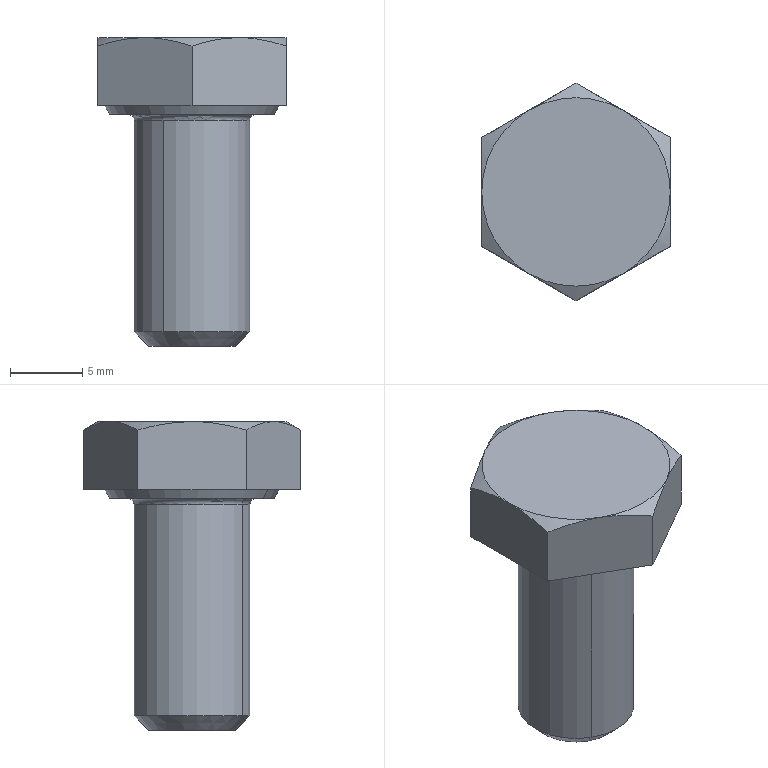Component | SolidWorks | GB_T5781-2000[HexHeadBoltFullThreadGradeCM8_16]-11 | 1 solid | 24 faces | box 13 x 15.01 x 21.3 mm | volume 1544 mm3 | cone 10 | plane 10 | cylinder 2 | torus 2 | commonest cylinder face diameters 8 x2
build123d program:
from build123d import *

# Parameters (mm, degrees)
BASE_EXTRUDE_DEPTH = 5.3
CHAMFER_2_SIZE     = 1


with BuildPart() as part:
    # Sketch1 → Base-Extrude (new body)
    with BuildSketch(Plane(origin=(0, 0, 0), x_dir=(0, 0, -1), z_dir=(1, 0, 0))):
        Polygon((6.5, 3.753), (6.5, -3.753), (0, -7.506), (-6.5, -3.753), (-6.5, 3.753), (0, 7.506), align=None)
    extrude(amount=BASE_EXTRUDE_DEPTH)

    # Sketch2 → Revolve1 (revolve)
    with BuildSketch(Plane.XY, mode=Mode.PRIVATE) as revolve1_sk:
        Polygon((0, 0), (21.3, 0), (21.3, 2.917), (21.3, 4), (5.3, 4), (0, 4), align=None)
    revolve(revolve1_sk.sketch.rotate(Axis((0, 0, 0), (-1, 0, 0)), 90), axis=Axis((0, 0, 0), (-1, 0, 0)))

    # Sketch3 → Cut-Revolve1 (revolve, cut)
    with BuildSketch(Plane.XY):
        Polygon((0, 6.5), (3.467, 12.506), (3.467, 17.506), (-10, 17.506), (-10, 6.5), align=None)
    revolve(axis=Axis((0, 0, 0), (1, 0, 0)), mode=Mode.SUBTRACT)

    # Sketch5 → Cut-Revolve2 (revolve, cut)
    with BuildSketch(Plane.XY):
        Polygon((5.3, 6.5), (1.833, 12.506), (1.833, 17.506), (11.833, 17.506), (11.833, 6.5), align=None)
    revolve(axis=Axis((0, 0, 0), (1, 0, 0)), mode=Mode.SUBTRACT)

    # Sketch4 → Cut-Revolve3 (revolve, cut)
    with BuildSketch(Plane.XY, mode=Mode.PRIVATE) as cut_revolve3_sk:
        Polygon((5.3, 5.677), (4.7, 6.024), (4.7, 17.506), (5.3, 17.506), align=None)
    revolve(cut_revolve3_sk.sketch.rotate(Axis((0, 0, 0), (1, 0, 0)), 90), axis=Axis((0, 0, 0), (1, 0, 0)), mode=Mode.SUBTRACT)

    # Chamfer 2
    chamfer_2_edges = [part.edges().sort_by_distance(p)[0] for p in [
        (21.3, 0, 4),
    ]]
    chamfer(chamfer_2_edges, length=CHAMFER_2_SIZE)

    # Sketch9 → Revolve1_2 (revolve)
    with BuildSketch(Plane.XY, mode=Mode.PRIVATE) as revolve1_2_sk:
        with BuildLine():
            Line((5.3, 4.4), (5.3, 4))
            Line((5.3, 4), (5.7, 4))
            ThreePointArc((5.7, 4), (5.417, 4.117), (5.3, 4.4))
        make_face()
    revolve(revolve1_2_sk.sketch.rotate(Axis((0, 0, 0), (1, 0, 0)), 90), axis=Axis((0, 0, 0), (1, 0, 0)))


solid = part.part

# Placed as in the assembly
solid = solid.moved(Location((24.99, 1.047, 168.3), (0, 90, 0)))
STEP:
#1=CARTESIAN_POINT('',(0.9051,-0.09515,6.402));
#2=VERTEX_POINT('',#1);
#3=CARTESIAN_POINT('',(1.063,0.1776,6.402));
#4=VERTEX_POINT('',#3);
#5=CARTESIAN_POINT('',(0.9839,0.04123,6.402));
#6=DIRECTION('',(-0.,-0.,1.));
#7=DIRECTION('',(-0.5,-0.866,-0.));
#8=AXIS2_PLACEMENT_3D('',#5,#6,#7);
#9=CIRCLE('',#8,0.1575);
#10=EDGE_CURVE('',#2,#4,#9,.T.);
#11=ORIENTED_EDGE('',*,*,#10,.F.);
#12=CARTESIAN_POINT('',(0.9051,-0.09515,5.827));
#13=VERTEX_POINT('',#12);
#14=CARTESIAN_POINT('',(0.9051,-0.09515,6.626));
#15=DIRECTION('',(0.,0.,-1.));
#16=VECTOR('',#15,39.37);
#17=LINE('',#14,#16);
#18=EDGE_CURVE('',#2,#13,#17,.T.);
#19=ORIENTED_EDGE('',*,*,#18,.T.);
#20=CARTESIAN_POINT('',(1.063,0.1776,5.827));
#21=VERTEX_POINT('',#20);
#22=CARTESIAN_POINT('',(0.9839,0.04123,5.827));
#23=DIRECTION('',(-0.,-0.,1.));
#24=DIRECTION('',(0.5,0.866,0.));
#25=AXIS2_PLACEMENT_3D('',#22,#23,#24);
#26=CIRCLE('',#25,0.1575);
#27=EDGE_CURVE('',#13,#21,#26,.T.);
#28=ORIENTED_EDGE('',*,*,#27,.T.);
#29=CARTESIAN_POINT('',(1.063,0.1776,6.626));
#30=DIRECTION('',(0.,0.,-1.));
#31=VECTOR('',#30,39.37);
#32=LINE('',#29,#31);
#33=EDGE_CURVE('',#4,#21,#32,.T.);
#34=ORIENTED_EDGE('',*,*,#33,.F.);
#35=EDGE_LOOP('',(#11,#19,#28,#34));
#36=FACE_OUTER_BOUND('',#35,.T.);
#37=CARTESIAN_POINT('',(0.9839,0.04123,6.626));
#38=DIRECTION('',(0.,0.,-1.));
#39=DIRECTION('',(0.5,0.866,0.));
#40=AXIS2_PLACEMENT_3D('',#37,#38,#39);
#41=CYLINDRICAL_SURFACE('',#40,0.1575);
#42=ADVANCED_FACE('',(#36),#41,.T.);
#43=CARTESIAN_POINT('',(1.043,0.1435,5.787));
#44=VERTEX_POINT('',#43);
#45=CARTESIAN_POINT('',(0.9248,-0.06106,5.787));
#46=VERTEX_POINT('',#45);
#47=CARTESIAN_POINT('',(0.9839,0.04123,5.787));
#48=DIRECTION('',(0.,0.,-1.));
#49=DIRECTION('',(0.5,0.866,0.));
#50=AXIS2_PLACEMENT_3D('',#47,#48,#49);
#51=CIRCLE('',#50,0.1181);
#52=EDGE_CURVE('',#44,#46,#51,.T.);
#53=ORIENTED_EDGE('',*,*,#52,.F.);
#54=CARTESIAN_POINT('',(1.043,0.1435,5.787));
#55=DIRECTION('',(0.3536,0.6124,0.7071));
#56=VECTOR('',#55,39.37);
#57=LINE('',#54,#56);
#58=EDGE_CURVE('',#44,#21,#57,.T.);
#59=ORIENTED_EDGE('',*,*,#58,.T.);
#60=ORIENTED_EDGE('',*,*,#27,.F.);
#61=CARTESIAN_POINT('',(0.9248,-0.06106,5.787));
#62=DIRECTION('',(-0.3536,-0.6124,0.7071));
#63=VECTOR('',#62,39.37);
#64=LINE('',#61,#63);
#65=EDGE_CURVE('',#46,#13,#64,.T.);
#66=ORIENTED_EDGE('',*,*,#65,.F.);
#67=EDGE_LOOP('',(#53,#59,#60,#66));
#68=FACE_OUTER_BOUND('',#67,.T.);
#69=CARTESIAN_POINT('',(0.9839,0.04123,5.787));
#70=DIRECTION('',(-0.,-0.,1.));
#71=DIRECTION('',(-0.5,-0.866,0.));
#72=AXIS2_PLACEMENT_3D('',#69,#70,#71);
#73=CONICAL_SURFACE('',#72,0.1181,0.7854);
#74=ADVANCED_FACE('',(#68),#73,.T.);
#75=CARTESIAN_POINT('',(1.07,0.1913,6.417));
#76=VERTEX_POINT('',#75);
#77=CARTESIAN_POINT('',(0.8972,-0.1088,6.417));
#78=VERTEX_POINT('',#77);
#79=CARTESIAN_POINT('',(0.9839,0.04123,6.417));
#80=DIRECTION('',(-0.,-0.,1.));
#81=DIRECTION('',(-0.5,-0.866,-0.));
#82=AXIS2_PLACEMENT_3D('',#79,#80,#81);
#83=CIRCLE('',#82,0.1732);
#84=EDGE_CURVE('',#76,#78,#83,.T.);
#85=ORIENTED_EDGE('',*,*,#84,.F.);
#86=CARTESIAN_POINT('',(1.07,0.1913,6.402));
#87=DIRECTION('',(0.866,-0.5,-0.));
#88=DIRECTION('',(0.5,0.866,0.));
#89=AXIS2_PLACEMENT_3D('',#86,#87,#88);
#90=CIRCLE('',#89,0.01575);
#91=EDGE_CURVE('',#76,#4,#90,.T.);
#92=ORIENTED_EDGE('',*,*,#91,.T.);
#93=CARTESIAN_POINT('',(0.9839,0.04123,6.402));
#94=DIRECTION('',(-0.,-0.,1.));
#95=DIRECTION('',(-0.5,-0.866,-0.));
#96=AXIS2_PLACEMENT_3D('',#93,#94,#95);
#97=CIRCLE('',#96,0.1575);
#98=EDGE_CURVE('',#4,#2,#97,.T.);
#99=ORIENTED_EDGE('',*,*,#98,.T.);
#100=CARTESIAN_POINT('',(0.8972,-0.1088,6.402));
#101=DIRECTION('',(-0.866,0.5,0.));
#102=DIRECTION('',(-0.5,-0.866,0.));
#103=AXIS2_PLACEMENT_3D('',#100,#101,#102);
#104=CIRCLE('',#103,0.01575);
#105=EDGE_CURVE('',#78,#2,#104,.T.);
#106=ORIENTED_EDGE('',*,*,#105,.F.);
#107=EDGE_LOOP('',(#85,#92,#99,#106));
#108=FACE_OUTER_BOUND('',#107,.T.);
#109=CARTESIAN_POINT('',(0.9839,0.04123,6.402));
#110=DIRECTION('',(-0.,-0.,1.));
#111=DIRECTION('',(-0.5,-0.866,-0.));
#112=AXIS2_PLACEMENT_3D('',#109,#110,#111);
#113=TOROIDAL_SURFACE('',#112,0.1732,0.01575);
#114=ADVANCED_FACE('',(#108),#113,.F.);
#115=CARTESIAN_POINT('',(0.8721,-0.1523,6.417));
#116=VERTEX_POINT('',#115);
#117=CARTESIAN_POINT('',(1.096,0.2348,6.417));
#118=VERTEX_POINT('',#117);
#119=CARTESIAN_POINT('',(0.9839,0.04123,6.417));
#120=DIRECTION('',(-0.,-0.,1.));
#121=DIRECTION('',(-0.5,-0.866,-0.));
#122=AXIS2_PLACEMENT_3D('',#119,#120,#121);
#123=CIRCLE('',#122,0.2235);
#124=EDGE_CURVE('',#116,#118,#123,.T.);
#125=ORIENTED_EDGE('',*,*,#124,.T.);
#126=CARTESIAN_POINT('',(1.102,0.2466,6.441));
#127=VERTEX_POINT('',#126);
#128=CARTESIAN_POINT('',(1.102,0.2466,6.441));
#129=DIRECTION('',(0.25,0.433,0.866));
#130=VECTOR('',#129,39.37);
#131=LINE('',#128,#130);
#132=EDGE_CURVE('',#118,#127,#131,.T.);
#133=ORIENTED_EDGE('',*,*,#132,.T.);
#134=CARTESIAN_POINT('',(0.8653,-0.1641,6.441));
#135=VERTEX_POINT('',#134);
#136=CARTESIAN_POINT('',(0.9839,0.04123,6.441));
#137=DIRECTION('',(-0.,-0.,1.));
#138=DIRECTION('',(-0.5,-0.866,-0.));
#139=AXIS2_PLACEMENT_3D('',#136,#137,#138);
#140=CIRCLE('',#139,0.2372);
#141=EDGE_CURVE('',#135,#127,#140,.T.);
#142=ORIENTED_EDGE('',*,*,#141,.F.);
#143=CARTESIAN_POINT('',(0.8653,-0.1641,6.441));
#144=DIRECTION('',(-0.25,-0.433,0.866));
#145=VECTOR('',#144,39.37);
#146=LINE('',#143,#145);
#147=EDGE_CURVE('',#116,#135,#146,.T.);
#148=ORIENTED_EDGE('',*,*,#147,.F.);
#149=EDGE_LOOP('',(#125,#133,#142,#148));
#150=FACE_OUTER_BOUND('',#149,.T.);
#151=CARTESIAN_POINT('',(0.9839,0.04123,6.441));
#152=DIRECTION('',(-0.,-0.,1.));
#153=DIRECTION('',(-0.5,-0.866,-0.));
#154=AXIS2_PLACEMENT_3D('',#151,#152,#153);
#155=CONICAL_SURFACE('',#154,0.2372,0.5236);
#156=ADVANCED_FACE('',(#150),#155,.T.);
#157=ORIENTED_EDGE('',*,*,#124,.F.);
#158=CARTESIAN_POINT('',(0.9839,0.04123,6.417));
#159=DIRECTION('',(-0.,-0.,1.));
#160=DIRECTION('',(-0.5,-0.866,-0.));
#161=AXIS2_PLACEMENT_3D('',#158,#159,#160);
#162=CIRCLE('',#161,0.2235);
#163=EDGE_CURVE('',#118,#116,#162,.T.);
#164=ORIENTED_EDGE('',*,*,#163,.F.);
#165=EDGE_LOOP('',(#157,#164));
#166=FACE_OUTER_BOUND('',#165,.T.);
#167=CARTESIAN_POINT('',(0.9839,0.04123,6.417));
#168=DIRECTION('',(-0.,-0.,1.));
#169=DIRECTION('',(-0.5,-0.866,-0.));
#170=AXIS2_PLACEMENT_3D('',#167,#168,#169);
#171=CIRCLE('',#170,0.1732);
#172=EDGE_CURVE('',#78,#76,#171,.T.);
#173=ORIENTED_EDGE('',*,*,#172,.T.);
#174=ORIENTED_EDGE('',*,*,#84,.T.);
#175=EDGE_LOOP('',(#173,#174));
#176=FACE_BOUND('',#175,.T.);
#177=CARTESIAN_POINT('',(1.24,-0.1065,6.417));
#178=DIRECTION('',(0.,0.,-1.));
#179=DIRECTION('',(0.5,0.866,0.));
#180=AXIS2_PLACEMENT_3D('',#177,#178,#179);
#181=PLANE('',#180);
#182=ADVANCED_FACE('',(#166,#176),#181,.T.);
#183=CARTESIAN_POINT('',(1.24,0.189,6.441));
#184=VERTEX_POINT('',#183);
#185=CARTESIAN_POINT('',(1.24,-0.1065,6.441));
#186=VERTEX_POINT('',#185);
#187=CARTESIAN_POINT('',(1.24,0.189,6.441));
#188=DIRECTION('',(0.,-1.,-0.));
#189=VECTOR('',#188,39.37);
#190=LINE('',#187,#189);
#191=EDGE_CURVE('',#184,#186,#190,.T.);
#192=ORIENTED_EDGE('',*,*,#191,.F.);
#193=CARTESIAN_POINT('',(1.24,0.189,6.603));
#194=VERTEX_POINT('',#193);
#195=CARTESIAN_POINT('',(1.24,0.189,6.417));
#196=DIRECTION('',(-0.,-0.,1.));
#197=VECTOR('',#196,39.37);
#198=LINE('',#195,#197);
#199=EDGE_CURVE('',#184,#194,#198,.T.);
#200=ORIENTED_EDGE('',*,*,#199,.T.);
#201=CARTESIAN_POINT('',(1.24,0.04123,6.626));
#202=VERTEX_POINT('',#201);
#203=CARTESIAN_POINT('',(1.24,0.04123,6.626));
#204=CARTESIAN_POINT('',(1.24,0.05377,6.626));
#205=CARTESIAN_POINT('',(1.24,0.06637,6.625));
#206=CARTESIAN_POINT('',(1.24,0.09128,6.623));
#207=CARTESIAN_POINT('',(1.24,0.1037,6.622));
#208=CARTESIAN_POINT('',(1.24,0.1406,6.616));
#209=CARTESIAN_POINT('',(1.24,0.1649,6.61));
#210=CARTESIAN_POINT('',(1.24,0.189,6.603));
#211=B_SPLINE_CURVE_WITH_KNOTS('',3,(#203,#204,#205,#206,#207,#208,#209,#210),.UNSPECIFIED.,.F.,.F.,(4,2,2,4),(0.003797,0.004743,0.005689,0.00758),.UNSPECIFIED.);
#212=EDGE_CURVE('',#202,#194,#211,.T.);
#213=ORIENTED_EDGE('',*,*,#212,.F.);
#214=CARTESIAN_POINT('',(1.24,-0.1065,6.603));
#215=VERTEX_POINT('',#214);
#216=CARTESIAN_POINT('',(1.24,-0.1065,6.603));
#217=CARTESIAN_POINT('',(1.24,-0.08235,6.61));
#218=CARTESIAN_POINT('',(1.24,-0.058,6.616));
#219=CARTESIAN_POINT('',(1.24,-0.008799,6.624));
#220=CARTESIAN_POINT('',(1.24,0.01606,6.626));
#221=CARTESIAN_POINT('',(1.24,0.04123,6.626));
#222=B_SPLINE_CURVE_WITH_KNOTS('',3,(#216,#217,#218,#219,#220,#221),.UNSPECIFIED.,.F.,.F.,(4,2,4),(0.00000024,0.001899,0.003797),.UNSPECIFIED.);
#223=EDGE_CURVE('',#215,#202,#222,.T.);
#224=ORIENTED_EDGE('',*,*,#223,.F.);
#225=CARTESIAN_POINT('',(1.24,-0.1065,6.417));
#226=DIRECTION('',(-0.,-0.,1.));
#227=VECTOR('',#226,39.37);
#228=LINE('',#225,#227);
#229=EDGE_CURVE('',#186,#215,#228,.T.);
#230=ORIENTED_EDGE('',*,*,#229,.F.);
#231=EDGE_LOOP('',(#192,#200,#213,#224,#230));
#232=FACE_OUTER_BOUND('',#231,.T.);
#233=CARTESIAN_POINT('',(1.24,0.189,6.417));
#234=DIRECTION('',(-1.,-0.,-0.));
#235=DIRECTION('',(-0.,1.,0.));
#236=AXIS2_PLACEMENT_3D('',#233,#234,#235);
#237=PLANE('',#236);
#238=ADVANCED_FACE('',(#232),#237,.F.);
#239=CARTESIAN_POINT('',(0.9839,-0.2543,6.441));
#240=VERTEX_POINT('',#239);
#241=CARTESIAN_POINT('',(1.24,-0.1065,6.441));
#242=DIRECTION('',(-0.866,-0.5,-0.));
#243=VECTOR('',#242,39.37);
#244=LINE('',#241,#243);
#245=EDGE_CURVE('',#186,#240,#244,.T.);
#246=ORIENTED_EDGE('',*,*,#245,.F.);
#247=ORIENTED_EDGE('',*,*,#229,.T.);
#248=CARTESIAN_POINT('',(1.112,-0.1804,6.626));
#249=VERTEX_POINT('',#248);
#250=CARTESIAN_POINT('',(1.112,-0.1804,6.626));
#251=CARTESIAN_POINT('',(1.123,-0.1741,6.626));
#252=CARTESIAN_POINT('',(1.134,-0.1678,6.625));
#253=CARTESIAN_POINT('',(1.155,-0.1554,6.623));
#254=CARTESIAN_POINT('',(1.166,-0.1492,6.622));
#255=CARTESIAN_POINT('',(1.198,-0.1307,6.616));
#256=CARTESIAN_POINT('',(1.219,-0.1186,6.61));
#257=CARTESIAN_POINT('',(1.24,-0.1065,6.603));
#258=B_SPLINE_CURVE_WITH_KNOTS('',3,(#250,#251,#252,#253,#254,#255,#256,#257),.UNSPECIFIED.,.F.,.F.,(4,2,2,4),(0.003797,0.004743,0.005689,0.00758),.UNSPECIFIED.);
#259=EDGE_CURVE('',#249,#215,#258,.T.);
#260=ORIENTED_EDGE('',*,*,#259,.F.);
#261=CARTESIAN_POINT('',(0.9839,-0.2543,6.603));
#262=VERTEX_POINT('',#261);
#263=CARTESIAN_POINT('',(0.9839,-0.2543,6.603));
#264=CARTESIAN_POINT('',(1.005,-0.2422,6.61));
#265=CARTESIAN_POINT('',(1.026,-0.23,6.616));
#266=CARTESIAN_POINT('',(1.068,-0.2054,6.624));
#267=CARTESIAN_POINT('',(1.09,-0.193,6.626));
#268=CARTESIAN_POINT('',(1.112,-0.1804,6.626));
#269=B_SPLINE_CURVE_WITH_KNOTS('',3,(#263,#264,#265,#266,#267,#268),.UNSPECIFIED.,.F.,.F.,(4,2,4),(0.00000024,0.001899,0.003797),.UNSPECIFIED.);
#270=EDGE_CURVE('',#262,#249,#269,.T.);
#271=ORIENTED_EDGE('',*,*,#270,.F.);
#272=CARTESIAN_POINT('',(0.9839,-0.2543,6.417));
#273=DIRECTION('',(-0.,-0.,1.));
#274=VECTOR('',#273,39.37);
#275=LINE('',#272,#274);
#276=EDGE_CURVE('',#240,#262,#275,.T.);
#277=ORIENTED_EDGE('',*,*,#276,.F.);
#278=EDGE_LOOP('',(#246,#247,#260,#271,#277));
#279=FACE_OUTER_BOUND('',#278,.T.);
#280=CARTESIAN_POINT('',(1.24,-0.1065,6.417));
#281=DIRECTION('',(-0.5,0.866,0.));
#282=DIRECTION('',(0.866,0.5,0.));
#283=AXIS2_PLACEMENT_3D('',#280,#281,#282);
#284=PLANE('',#283);
#285=ADVANCED_FACE('',(#279),#284,.F.);
#286=CARTESIAN_POINT('',(0.728,-0.1065,6.441));
#287=VERTEX_POINT('',#286);
#288=CARTESIAN_POINT('',(0.9839,-0.2543,6.441));
#289=DIRECTION('',(-0.866,0.5,0.));
#290=VECTOR('',#289,39.37);
#291=LINE('',#288,#290);
#292=EDGE_CURVE('',#240,#287,#291,.T.);
#293=ORIENTED_EDGE('',*,*,#292,.F.);
#294=ORIENTED_EDGE('',*,*,#276,.T.);
#295=CARTESIAN_POINT('',(0.8559,-0.1804,6.626));
#296=VERTEX_POINT('',#295);
#297=CARTESIAN_POINT('',(0.8559,-0.1804,6.626));
#298=CARTESIAN_POINT('',(0.8776,-0.1929,6.626));
#299=CARTESIAN_POINT('',(0.8995,-0.2056,6.624));
#300=CARTESIAN_POINT('',(0.9422,-0.2302,6.616));
#301=CARTESIAN_POINT('',(0.9632,-0.2423,6.61));
#302=CARTESIAN_POINT('',(0.9839,-0.2543,6.603));
#303=B_SPLINE_CURVE_WITH_KNOTS('',3,(#297,#298,#299,#300,#301,#302),.UNSPECIFIED.,.F.,.F.,(4,2,4),(0.01067,0.01257,0.01447),.UNSPECIFIED.);
#304=EDGE_CURVE('',#296,#262,#303,.T.);
#305=ORIENTED_EDGE('',*,*,#304,.F.);
#306=CARTESIAN_POINT('',(0.728,-0.1065,6.603));
#307=VERTEX_POINT('',#306);
#308=CARTESIAN_POINT('',(0.728,-0.1065,6.603));
#309=CARTESIAN_POINT('',(0.7488,-0.1185,6.61));
#310=CARTESIAN_POINT('',(0.7701,-0.1308,6.616));
#311=CARTESIAN_POINT('',(0.8128,-0.1555,6.624));
#312=CARTESIAN_POINT('',(0.8343,-0.1679,6.626));
#313=CARTESIAN_POINT('',(0.8559,-0.1804,6.626));
#314=B_SPLINE_CURVE_WITH_KNOTS('',3,(#308,#309,#310,#311,#312,#313),.UNSPECIFIED.,.F.,.F.,(4,2,4),(0.006874,0.008773,0.01067),.UNSPECIFIED.);
#315=EDGE_CURVE('',#307,#296,#314,.T.);
#316=ORIENTED_EDGE('',*,*,#315,.F.);
#317=CARTESIAN_POINT('',(0.728,-0.1065,6.417));
#318=DIRECTION('',(-0.,-0.,1.));
#319=VECTOR('',#318,39.37);
#320=LINE('',#317,#319);
#321=EDGE_CURVE('',#287,#307,#320,.T.);
#322=ORIENTED_EDGE('',*,*,#321,.F.);
#323=EDGE_LOOP('',(#293,#294,#305,#316,#322));
#324=FACE_OUTER_BOUND('',#323,.T.);
#325=CARTESIAN_POINT('',(0.9839,-0.2543,6.417));
#326=DIRECTION('',(0.5,0.866,0.));
#327=DIRECTION('',(0.866,-0.5,-0.));
#328=AXIS2_PLACEMENT_3D('',#325,#326,#327);
#329=PLANE('',#328);
#330=ADVANCED_FACE('',(#324),#329,.F.);
#331=CARTESIAN_POINT('',(0.728,0.189,6.441));
#332=VERTEX_POINT('',#331);
#333=CARTESIAN_POINT('',(0.728,0.189,6.441));
#334=DIRECTION('',(-0.,1.,0.));
#335=VECTOR('',#334,39.37);
#336=LINE('',#333,#335);
#337=EDGE_CURVE('',#287,#332,#336,.T.);
#338=ORIENTED_EDGE('',*,*,#337,.F.);
#339=ORIENTED_EDGE('',*,*,#321,.T.);
#340=CARTESIAN_POINT('',(0.728,0.04123,6.626));
#341=VERTEX_POINT('',#340);
#342=CARTESIAN_POINT('',(0.728,0.04123,6.626));
#343=CARTESIAN_POINT('',(0.728,0.02869,6.626));
#344=CARTESIAN_POINT('',(0.728,0.0161,6.625));
#345=CARTESIAN_POINT('',(0.728,-0.008818,6.623));
#346=CARTESIAN_POINT('',(0.728,-0.02119,6.622));
#347=CARTESIAN_POINT('',(0.728,-0.0581,6.616));
#348=CARTESIAN_POINT('',(0.728,-0.08241,6.61));
#349=CARTESIAN_POINT('',(0.728,-0.1065,6.603));
#350=B_SPLINE_CURVE_WITH_KNOTS('',3,(#342,#343,#344,#345,#346,#347,#348,#349),.UNSPECIFIED.,.F.,.F.,(4,2,2,4),(0.003797,0.004743,0.005689,0.00758),.UNSPECIFIED.);
#351=EDGE_CURVE('',#341,#307,#350,.T.);
#352=ORIENTED_EDGE('',*,*,#351,.F.);
#353=CARTESIAN_POINT('',(0.728,0.189,6.603));
#354=VERTEX_POINT('',#353);
#355=CARTESIAN_POINT('',(0.728,0.189,6.603));
#356=CARTESIAN_POINT('',(0.728,0.1648,6.61));
#357=CARTESIAN_POINT('',(0.728,0.1405,6.616));
#358=CARTESIAN_POINT('',(0.728,0.09126,6.624));
#359=CARTESIAN_POINT('',(0.728,0.0664,6.626));
#360=CARTESIAN_POINT('',(0.728,0.04123,6.626));
#361=B_SPLINE_CURVE_WITH_KNOTS('',3,(#355,#356,#357,#358,#359,#360),.UNSPECIFIED.,.F.,.F.,(4,2,4),(0.00000024,0.001899,0.003797),.UNSPECIFIED.);
#362=EDGE_CURVE('',#354,#341,#361,.T.);
#363=ORIENTED_EDGE('',*,*,#362,.F.);
#364=CARTESIAN_POINT('',(0.728,0.189,6.417));
#365=DIRECTION('',(-0.,-0.,1.));
#366=VECTOR('',#365,39.37);
#367=LINE('',#364,#366);
#368=EDGE_CURVE('',#332,#354,#367,.T.);
#369=ORIENTED_EDGE('',*,*,#368,.F.);
#370=EDGE_LOOP('',(#338,#339,#352,#363,#369));
#371=FACE_OUTER_BOUND('',#370,.T.);
#372=CARTESIAN_POINT('',(0.728,0.189,6.417));
#373=DIRECTION('',(1.,0.,0.));
#374=DIRECTION('',(0.,-1.,-0.));
#375=AXIS2_PLACEMENT_3D('',#372,#373,#374);
#376=PLANE('',#375);
#377=ADVANCED_FACE('',(#371),#376,.F.);
#378=CARTESIAN_POINT('',(0.9839,0.3367,6.441));
#379=VERTEX_POINT('',#378);
#380=CARTESIAN_POINT('',(0.9839,0.3367,6.441));
#381=DIRECTION('',(0.866,0.5,0.));
#382=VECTOR('',#381,39.37);
#383=LINE('',#380,#382);
#384=EDGE_CURVE('',#332,#379,#383,.T.);
#385=ORIENTED_EDGE('',*,*,#384,.F.);
#386=ORIENTED_EDGE('',*,*,#368,.T.);
#387=CARTESIAN_POINT('',(0.8559,0.2629,6.626));
#388=VERTEX_POINT('',#387);
#389=CARTESIAN_POINT('',(0.8559,0.2629,6.626));
#390=CARTESIAN_POINT('',(0.845,0.2566,6.626));
#391=CARTESIAN_POINT('',(0.8341,0.2503,6.625));
#392=CARTESIAN_POINT('',(0.8126,0.2378,6.623));
#393=CARTESIAN_POINT('',(0.8018,0.2316,6.622));
#394=CARTESIAN_POINT('',(0.7699,0.2132,6.616));
#395=CARTESIAN_POINT('',(0.7488,0.201,6.61));
#396=CARTESIAN_POINT('',(0.728,0.189,6.603));
#397=B_SPLINE_CURVE_WITH_KNOTS('',3,(#389,#390,#391,#392,#393,#394,#395,#396),.UNSPECIFIED.,.F.,.F.,(4,2,2,4),(0.003797,0.004743,0.005689,0.00758),.UNSPECIFIED.);
#398=EDGE_CURVE('',#388,#354,#397,.T.);
#399=ORIENTED_EDGE('',*,*,#398,.F.);
#400=CARTESIAN_POINT('',(0.9839,0.3367,6.603));
#401=VERTEX_POINT('',#400);
#402=CARTESIAN_POINT('',(0.9839,0.3367,6.603));
#403=CARTESIAN_POINT('',(0.9629,0.3246,6.61));
#404=CARTESIAN_POINT('',(0.9418,0.3125,6.616));
#405=CARTESIAN_POINT('',(0.8992,0.2879,6.624));
#406=CARTESIAN_POINT('',(0.8777,0.2754,6.626));
#407=CARTESIAN_POINT('',(0.8559,0.2629,6.626));
#408=B_SPLINE_CURVE_WITH_KNOTS('',3,(#402,#403,#404,#405,#406,#407),.UNSPECIFIED.,.F.,.F.,(4,2,4),(0.00000024,0.001899,0.003797),.UNSPECIFIED.);
#409=EDGE_CURVE('',#401,#388,#408,.T.);
#410=ORIENTED_EDGE('',*,*,#409,.F.);
#411=CARTESIAN_POINT('',(0.9839,0.3367,6.417));
#412=DIRECTION('',(-0.,-0.,1.));
#413=VECTOR('',#412,39.37);
#414=LINE('',#411,#413);
#415=EDGE_CURVE('',#379,#401,#414,.T.);
#416=ORIENTED_EDGE('',*,*,#415,.F.);
#417=EDGE_LOOP('',(#385,#386,#399,#410,#416));
#418=FACE_OUTER_BOUND('',#417,.T.);
#419=CARTESIAN_POINT('',(0.9839,0.3367,6.417));
#420=DIRECTION('',(0.5,-0.866,-0.));
#421=DIRECTION('',(-0.866,-0.5,-0.));
#422=AXIS2_PLACEMENT_3D('',#419,#420,#421);
#423=PLANE('',#422);
#424=ADVANCED_FACE('',(#418),#423,.F.);
#425=CARTESIAN_POINT('',(1.24,0.189,6.441));
#426=DIRECTION('',(0.866,-0.5,-0.));
#427=VECTOR('',#426,39.37);
#428=LINE('',#425,#427);
#429=EDGE_CURVE('',#379,#184,#428,.T.);
#430=ORIENTED_EDGE('',*,*,#429,.F.);
#431=ORIENTED_EDGE('',*,*,#415,.T.);
#432=CARTESIAN_POINT('',(1.112,0.2629,6.626));
#433=VERTEX_POINT('',#432);
#434=CARTESIAN_POINT('',(1.112,0.2629,6.626));
#435=CARTESIAN_POINT('',(1.09,0.2753,6.626));
#436=CARTESIAN_POINT('',(1.069,0.2877,6.624));
#437=CARTESIAN_POINT('',(1.026,0.3124,6.616));
#438=CARTESIAN_POINT('',(1.005,0.3247,6.61));
#439=CARTESIAN_POINT('',(0.9839,0.3367,6.603));
#440=B_SPLINE_CURVE_WITH_KNOTS('',3,(#434,#435,#436,#437,#438,#439),.UNSPECIFIED.,.F.,.F.,(4,2,4),(0.02294,0.02484,0.02674),.UNSPECIFIED.);
#441=EDGE_CURVE('',#433,#401,#440,.T.);
#442=ORIENTED_EDGE('',*,*,#441,.F.);
#443=CARTESIAN_POINT('',(1.24,0.189,6.603));
#444=CARTESIAN_POINT('',(1.219,0.2009,6.61));
#445=CARTESIAN_POINT('',(1.198,0.213,6.616));
#446=CARTESIAN_POINT('',(1.155,0.2377,6.624));
#447=CARTESIAN_POINT('',(1.133,0.2503,6.626));
#448=CARTESIAN_POINT('',(1.112,0.2629,6.626));
#449=B_SPLINE_CURVE_WITH_KNOTS('',3,(#443,#444,#445,#446,#447,#448),.UNSPECIFIED.,.F.,.F.,(4,2,4),(0.01914,0.02104,0.02294),.UNSPECIFIED.);
#450=EDGE_CURVE('',#194,#433,#449,.T.);
#451=ORIENTED_EDGE('',*,*,#450,.F.);
#452=ORIENTED_EDGE('',*,*,#199,.F.);
#453=EDGE_LOOP('',(#430,#431,#442,#451,#452));
#454=FACE_OUTER_BOUND('',#453,.T.);
#455=CARTESIAN_POINT('',(1.24,0.189,6.417));
#456=DIRECTION('',(-0.5,-0.866,-0.));
#457=DIRECTION('',(-0.866,0.5,0.));
#458=AXIS2_PLACEMENT_3D('',#455,#456,#457);
#459=PLANE('',#458);
#460=ADVANCED_FACE('',(#454),#459,.F.);
#461=ORIENTED_EDGE('',*,*,#409,.T.);
#462=CARTESIAN_POINT('',(0.9839,0.04123,6.626));
#463=DIRECTION('',(0.,0.,-1.));
#464=DIRECTION('',(0.5,0.866,0.));
#465=AXIS2_PLACEMENT_3D('',#462,#463,#464);
#466=CIRCLE('',#465,0.2559);
#467=EDGE_CURVE('',#388,#433,#466,.T.);
#468=ORIENTED_EDGE('',*,*,#467,.T.);
#469=ORIENTED_EDGE('',*,*,#441,.T.);
#470=EDGE_LOOP('',(#461,#468,#469));
#471=FACE_OUTER_BOUND('',#470,.T.);
#472=CARTESIAN_POINT('',(0.9839,0.04123,6.626));
#473=DIRECTION('',(0.,0.,-1.));
#474=DIRECTION('',(0.5,0.866,0.));
#475=AXIS2_PLACEMENT_3D('',#472,#473,#474);
#476=CONICAL_SURFACE('',#475,0.2559,1.047);
#477=ADVANCED_FACE('',(#471),#476,.T.);
#478=ORIENTED_EDGE('',*,*,#362,.T.);
#479=CARTESIAN_POINT('',(0.9839,0.04123,6.626));
#480=DIRECTION('',(0.,0.,-1.));
#481=DIRECTION('',(0.5,0.866,0.));
#482=AXIS2_PLACEMENT_3D('',#479,#480,#481);
#483=CIRCLE('',#482,0.2559);
#484=EDGE_CURVE('',#341,#388,#483,.T.);
#485=ORIENTED_EDGE('',*,*,#484,.T.);
#486=ORIENTED_EDGE('',*,*,#398,.T.);
#487=EDGE_LOOP('',(#478,#485,#486));
#488=FACE_OUTER_BOUND('',#487,.T.);
#489=CARTESIAN_POINT('',(0.9839,0.04123,6.626));
#490=DIRECTION('',(0.,0.,-1.));
#491=DIRECTION('',(0.5,0.866,0.));
#492=AXIS2_PLACEMENT_3D('',#489,#490,#491);
#493=CONICAL_SURFACE('',#492,0.2559,1.047);
#494=ADVANCED_FACE('',(#488),#493,.T.);
#495=ORIENTED_EDGE('',*,*,#315,.T.);
#496=CARTESIAN_POINT('',(0.9839,0.04123,6.626));
#497=DIRECTION('',(0.,0.,-1.));
#498=DIRECTION('',(0.5,0.866,0.));
#499=AXIS2_PLACEMENT_3D('',#496,#497,#498);
#500=CIRCLE('',#499,0.2559);
#501=EDGE_CURVE('',#296,#341,#500,.T.);
#502=ORIENTED_EDGE('',*,*,#501,.T.);
#503=ORIENTED_EDGE('',*,*,#351,.T.);
#504=EDGE_LOOP('',(#495,#502,#503));
#505=FACE_OUTER_BOUND('',#504,.T.);
#506=CARTESIAN_POINT('',(0.9839,0.04123,6.626));
#507=DIRECTION('',(0.,0.,-1.));
#508=DIRECTION('',(0.5,0.866,0.));
#509=AXIS2_PLACEMENT_3D('',#506,#507,#508);
#510=CONICAL_SURFACE('',#509,0.2559,1.047);
#511=ADVANCED_FACE('',(#505),#510,.T.);
#512=ORIENTED_EDGE('',*,*,#304,.T.);
#513=ORIENTED_EDGE('',*,*,#270,.T.);
#514=CARTESIAN_POINT('',(0.9839,0.04123,6.626));
#515=DIRECTION('',(-0.,-0.,1.));
#516=DIRECTION('',(-0.5,-0.866,-0.));
#517=AXIS2_PLACEMENT_3D('',#514,#515,#516);
#518=CIRCLE('',#517,0.2559);
#519=EDGE_CURVE('',#296,#249,#518,.T.);
#520=ORIENTED_EDGE('',*,*,#519,.F.);
#521=EDGE_LOOP('',(#512,#513,#520));
#522=FACE_OUTER_BOUND('',#521,.T.);
#523=CARTESIAN_POINT('',(0.9839,0.04123,6.626));
#524=DIRECTION('',(0.,0.,-1.));
#525=DIRECTION('',(0.5,0.866,0.));
#526=AXIS2_PLACEMENT_3D('',#523,#524,#525);
#527=CONICAL_SURFACE('',#526,0.2559,1.047);
#528=ADVANCED_FACE('',(#522),#527,.T.);
#529=ORIENTED_EDGE('',*,*,#259,.T.);
#530=ORIENTED_EDGE('',*,*,#223,.T.);
#531=CARTESIAN_POINT('',(0.9839,0.04123,6.626));
#532=DIRECTION('',(0.,0.,-1.));
#533=DIRECTION('',(0.5,0.866,0.));
#534=AXIS2_PLACEMENT_3D('',#531,#532,#533);
#535=CIRCLE('',#534,0.2559);
#536=EDGE_CURVE('',#202,#249,#535,.T.);
#537=ORIENTED_EDGE('',*,*,#536,.T.);
#538=EDGE_LOOP('',(#529,#530,#537));
#539=FACE_OUTER_BOUND('',#538,.T.);
#540=CARTESIAN_POINT('',(0.9839,0.04123,6.626));
#541=DIRECTION('',(0.,0.,-1.));
#542=DIRECTION('',(0.5,0.866,0.));
#543=AXIS2_PLACEMENT_3D('',#540,#541,#542);
#544=CONICAL_SURFACE('',#543,0.2559,1.047);
#545=ADVANCED_FACE('',(#539),#544,.T.);
#546=ORIENTED_EDGE('',*,*,#212,.T.);
#547=ORIENTED_EDGE('',*,*,#450,.T.);
#548=CARTESIAN_POINT('',(0.9839,0.04123,6.626));
#549=DIRECTION('',(0.,0.,-1.));
#550=DIRECTION('',(0.5,0.866,0.));
#551=AXIS2_PLACEMENT_3D('',#548,#549,#550);
#552=CIRCLE('',#551,0.2559);
#553=EDGE_CURVE('',#433,#202,#552,.T.);
#554=ORIENTED_EDGE('',*,*,#553,.T.);
#555=EDGE_LOOP('',(#546,#547,#554));
#556=FACE_OUTER_BOUND('',#555,.T.);
#557=CARTESIAN_POINT('',(0.9839,0.04123,6.626));
#558=DIRECTION('',(0.,0.,-1.));
#559=DIRECTION('',(0.5,0.866,0.));
#560=AXIS2_PLACEMENT_3D('',#557,#558,#559);
#561=CONICAL_SURFACE('',#560,0.2559,1.047);
#562=ADVANCED_FACE('',(#556),#561,.T.);
#563=ORIENTED_EDGE('',*,*,#553,.F.);
#564=ORIENTED_EDGE('',*,*,#467,.F.);
#565=ORIENTED_EDGE('',*,*,#484,.F.);
#566=ORIENTED_EDGE('',*,*,#501,.F.);
#567=ORIENTED_EDGE('',*,*,#519,.T.);
#568=ORIENTED_EDGE('',*,*,#536,.F.);
#569=EDGE_LOOP('',(#563,#564,#565,#566,#567,#568));
#570=FACE_OUTER_BOUND('',#569,.T.);
#571=CARTESIAN_POINT('',(1.24,-0.1065,6.626));
#572=DIRECTION('',(0.,0.,-1.));
#573=DIRECTION('',(0.5,0.866,0.));
#574=AXIS2_PLACEMENT_3D('',#571,#572,#573);
#575=PLANE('',#574);
#576=ADVANCED_FACE('',(#570),#575,.F.);
#577=ORIENTED_EDGE('',*,*,#141,.T.);
#578=CARTESIAN_POINT('',(0.9839,0.04123,6.441));
#579=DIRECTION('',(-0.,-0.,1.));
#580=DIRECTION('',(-0.5,-0.866,-0.));
#581=AXIS2_PLACEMENT_3D('',#578,#579,#580);
#582=CIRCLE('',#581,0.2372);
#583=EDGE_CURVE('',#127,#135,#582,.T.);
#584=ORIENTED_EDGE('',*,*,#583,.T.);
#585=EDGE_LOOP('',(#577,#584));
#586=FACE_BOUND('',#585,.T.);
#587=ORIENTED_EDGE('',*,*,#191,.T.);
#588=ORIENTED_EDGE('',*,*,#245,.T.);
#589=ORIENTED_EDGE('',*,*,#292,.T.);
#590=ORIENTED_EDGE('',*,*,#337,.T.);
#591=ORIENTED_EDGE('',*,*,#384,.T.);
#592=ORIENTED_EDGE('',*,*,#429,.T.);
#593=EDGE_LOOP('',(#587,#588,#589,#590,#591,#592));
#594=FACE_OUTER_BOUND('',#593,.T.);
#595=CARTESIAN_POINT('',(1.189,-0.07734,6.441));
#596=DIRECTION('',(0.,0.,-1.));
#597=DIRECTION('',(0.5,0.866,0.));
#598=AXIS2_PLACEMENT_3D('',#595,#596,#597);
#599=PLANE('',#598);
#600=ADVANCED_FACE('',(#586,#594),#599,.T.);
#601=ORIENTED_EDGE('',*,*,#132,.F.);
#602=ORIENTED_EDGE('',*,*,#163,.T.);
#603=ORIENTED_EDGE('',*,*,#147,.T.);
#604=ORIENTED_EDGE('',*,*,#583,.F.);
#605=EDGE_LOOP('',(#601,#602,#603,#604));
#606=FACE_OUTER_BOUND('',#605,.T.);
#607=CARTESIAN_POINT('',(0.9839,0.04123,6.441));
#608=DIRECTION('',(-0.,-0.,1.));
#609=DIRECTION('',(-0.5,-0.866,-0.));
#610=AXIS2_PLACEMENT_3D('',#607,#608,#609);
#611=CONICAL_SURFACE('',#610,0.2372,0.5236);
#612=ADVANCED_FACE('',(#606),#611,.T.);
#613=ORIENTED_EDGE('',*,*,#91,.F.);
#614=ORIENTED_EDGE('',*,*,#172,.F.);
#615=ORIENTED_EDGE('',*,*,#105,.T.);
#616=ORIENTED_EDGE('',*,*,#10,.T.);
#617=EDGE_LOOP('',(#613,#614,#615,#616));
#618=FACE_OUTER_BOUND('',#617,.T.);
#619=CARTESIAN_POINT('',(0.9839,0.04123,6.402));
#620=DIRECTION('',(-0.,-0.,1.));
#621=DIRECTION('',(-0.5,-0.866,-0.));
#622=AXIS2_PLACEMENT_3D('',#619,#620,#621);
#623=TOROIDAL_SURFACE('',#622,0.1732,0.01575);
#624=ADVANCED_FACE('',(#618),#623,.F.);
#625=CARTESIAN_POINT('',(0.9839,0.04123,5.787));
#626=DIRECTION('',(0.,0.,-1.));
#627=DIRECTION('',(0.5,0.866,0.));
#628=AXIS2_PLACEMENT_3D('',#625,#626,#627);
#629=CIRCLE('',#628,0.1181);
#630=EDGE_CURVE('',#46,#44,#629,.T.);
#631=ORIENTED_EDGE('',*,*,#630,.T.);
#632=ORIENTED_EDGE('',*,*,#52,.T.);
#633=EDGE_LOOP('',(#631,#632));
#634=FACE_OUTER_BOUND('',#633,.T.);
#635=CARTESIAN_POINT('',(0.9839,0.04123,5.787));
#636=DIRECTION('',(0.,0.,-1.));
#637=DIRECTION('',(0.5,0.866,0.));
#638=AXIS2_PLACEMENT_3D('',#635,#636,#637);
#639=PLANE('',#638);
#640=ADVANCED_FACE('',(#634),#639,.T.);
#641=ORIENTED_EDGE('',*,*,#58,.F.);
#642=ORIENTED_EDGE('',*,*,#630,.F.);
#643=ORIENTED_EDGE('',*,*,#65,.T.);
#644=CARTESIAN_POINT('',(0.9839,0.04123,5.827));
#645=DIRECTION('',(-0.,-0.,1.));
#646=DIRECTION('',(0.5,0.866,0.));
#647=AXIS2_PLACEMENT_3D('',#644,#645,#646);
#648=CIRCLE('',#647,0.1575);
#649=EDGE_CURVE('',#21,#13,#648,.T.);
#650=ORIENTED_EDGE('',*,*,#649,.F.);
#651=EDGE_LOOP('',(#641,#642,#643,#650));
#652=FACE_OUTER_BOUND('',#651,.T.);
#653=CARTESIAN_POINT('',(0.9839,0.04123,5.787));
#654=DIRECTION('',(-0.,-0.,1.));
#655=DIRECTION('',(-0.5,-0.866,0.));
#656=AXIS2_PLACEMENT_3D('',#653,#654,#655);
#657=CONICAL_SURFACE('',#656,0.1181,0.7854);
#658=ADVANCED_FACE('',(#652),#657,.T.);
#659=ORIENTED_EDGE('',*,*,#18,.F.);
#660=ORIENTED_EDGE('',*,*,#98,.F.);
#661=ORIENTED_EDGE('',*,*,#33,.T.);
#662=ORIENTED_EDGE('',*,*,#649,.T.);
#663=EDGE_LOOP('',(#659,#660,#661,#662));
#664=FACE_OUTER_BOUND('',#663,.T.);
#665=CARTESIAN_POINT('',(0.9839,0.04123,6.626));
#666=DIRECTION('',(0.,0.,-1.));
#667=DIRECTION('',(0.5,0.866,0.));
#668=AXIS2_PLACEMENT_3D('',#665,#666,#667);
#669=CYLINDRICAL_SURFACE('',#668,0.1575);
#670=ADVANCED_FACE('',(#664),#669,.T.);
#671=CLOSED_SHELL('',(#42,#74,#114,#156,#182,#238,#285,#330,#377,#424,#460,#477,#494,#511,#528,#545,#562,#576,#600,#612,#624,#640,#658,#670));
#672=MANIFOLD_SOLID_BREP('',#671);
#673=CARTESIAN_POINT('',(0.,0.,0.));
#674=DIRECTION('',(0.,0.,1.));
#675=DIRECTION('',(1.,0.,0.));
#676=AXIS2_PLACEMENT_3D('',#673,#674,#675);
#677=(LENGTH_UNIT()NAMED_UNIT(*)SI_UNIT($,.METRE.));
#678=LENGTH_MEASURE_WITH_UNIT(LENGTH_MEASURE(0.0254),#677);
#679=DIMENSIONAL_EXPONENTS(1.,0.,0.,0.,0.,0.,0.);
#680=(CONVERSION_BASED_UNIT('',#678)LENGTH_UNIT()NAMED_UNIT(#679));
#681=UNCERTAINTY_MEASURE_WITH_UNIT(LENGTH_MEASURE(0.00001),#680,'','');
#682=(NAMED_UNIT(*)PLANE_ANGLE_UNIT()SI_UNIT($,.RADIAN.));
#683=(NAMED_UNIT(*)SI_UNIT($,.STERADIAN.)SOLID_ANGLE_UNIT());
#684=(GEOMETRIC_REPRESENTATION_CONTEXT(3)GLOBAL_UNCERTAINTY_ASSIGNED_CONTEXT((#681))GLOBAL_UNIT_ASSIGNED_CONTEXT((#680,#682,#683))REPRESENTATION_CONTEXT('',''));
#685=ADVANCED_BREP_SHAPE_REPRESENTATION('',(#672,#676),#684);
#686=COLOUR_RGB('',0.7922,0.8196,0.9333);
#687=FILL_AREA_STYLE_COLOUR('',#686);
#688=FILL_AREA_STYLE('',(#687));
#689=SURFACE_STYLE_FILL_AREA(#688);
#690=SURFACE_SIDE_STYLE('',(#689));
#691=SURFACE_STYLE_USAGE(.BOTH.,#690);
#692=PRESENTATION_STYLE_ASSIGNMENT((#691));
#693=STYLED_ITEM('',(#692),#672);
#694=(LENGTH_UNIT()NAMED_UNIT(*)SI_UNIT($,.METRE.));
#695=LENGTH_MEASURE_WITH_UNIT(LENGTH_MEASURE(0.0254),#694);
#696=DIMENSIONAL_EXPONENTS(1.,0.,0.,0.,0.,0.,0.);
#697=(CONVERSION_BASED_UNIT('',#695)LENGTH_UNIT()NAMED_UNIT(#696));
#698=UNCERTAINTY_MEASURE_WITH_UNIT(LENGTH_MEASURE(0.00001),#697,'','');
#699=(NAMED_UNIT(*)PLANE_ANGLE_UNIT()SI_UNIT($,.RADIAN.));
#700=(NAMED_UNIT(*)SI_UNIT($,.STERADIAN.)SOLID_ANGLE_UNIT());
#701=(GEOMETRIC_REPRESENTATION_CONTEXT(3)GLOBAL_UNCERTAINTY_ASSIGNED_CONTEXT((#698))GLOBAL_UNIT_ASSIGNED_CONTEXT((#697,#699,#700))REPRESENTATION_CONTEXT('',''));
#702=MECHANICAL_DESIGN_GEOMETRIC_PRESENTATION_REPRESENTATION('',(#693),#701);
#703=PRESENTATION_LAYER_ASSIGNMENT('','',(#693));